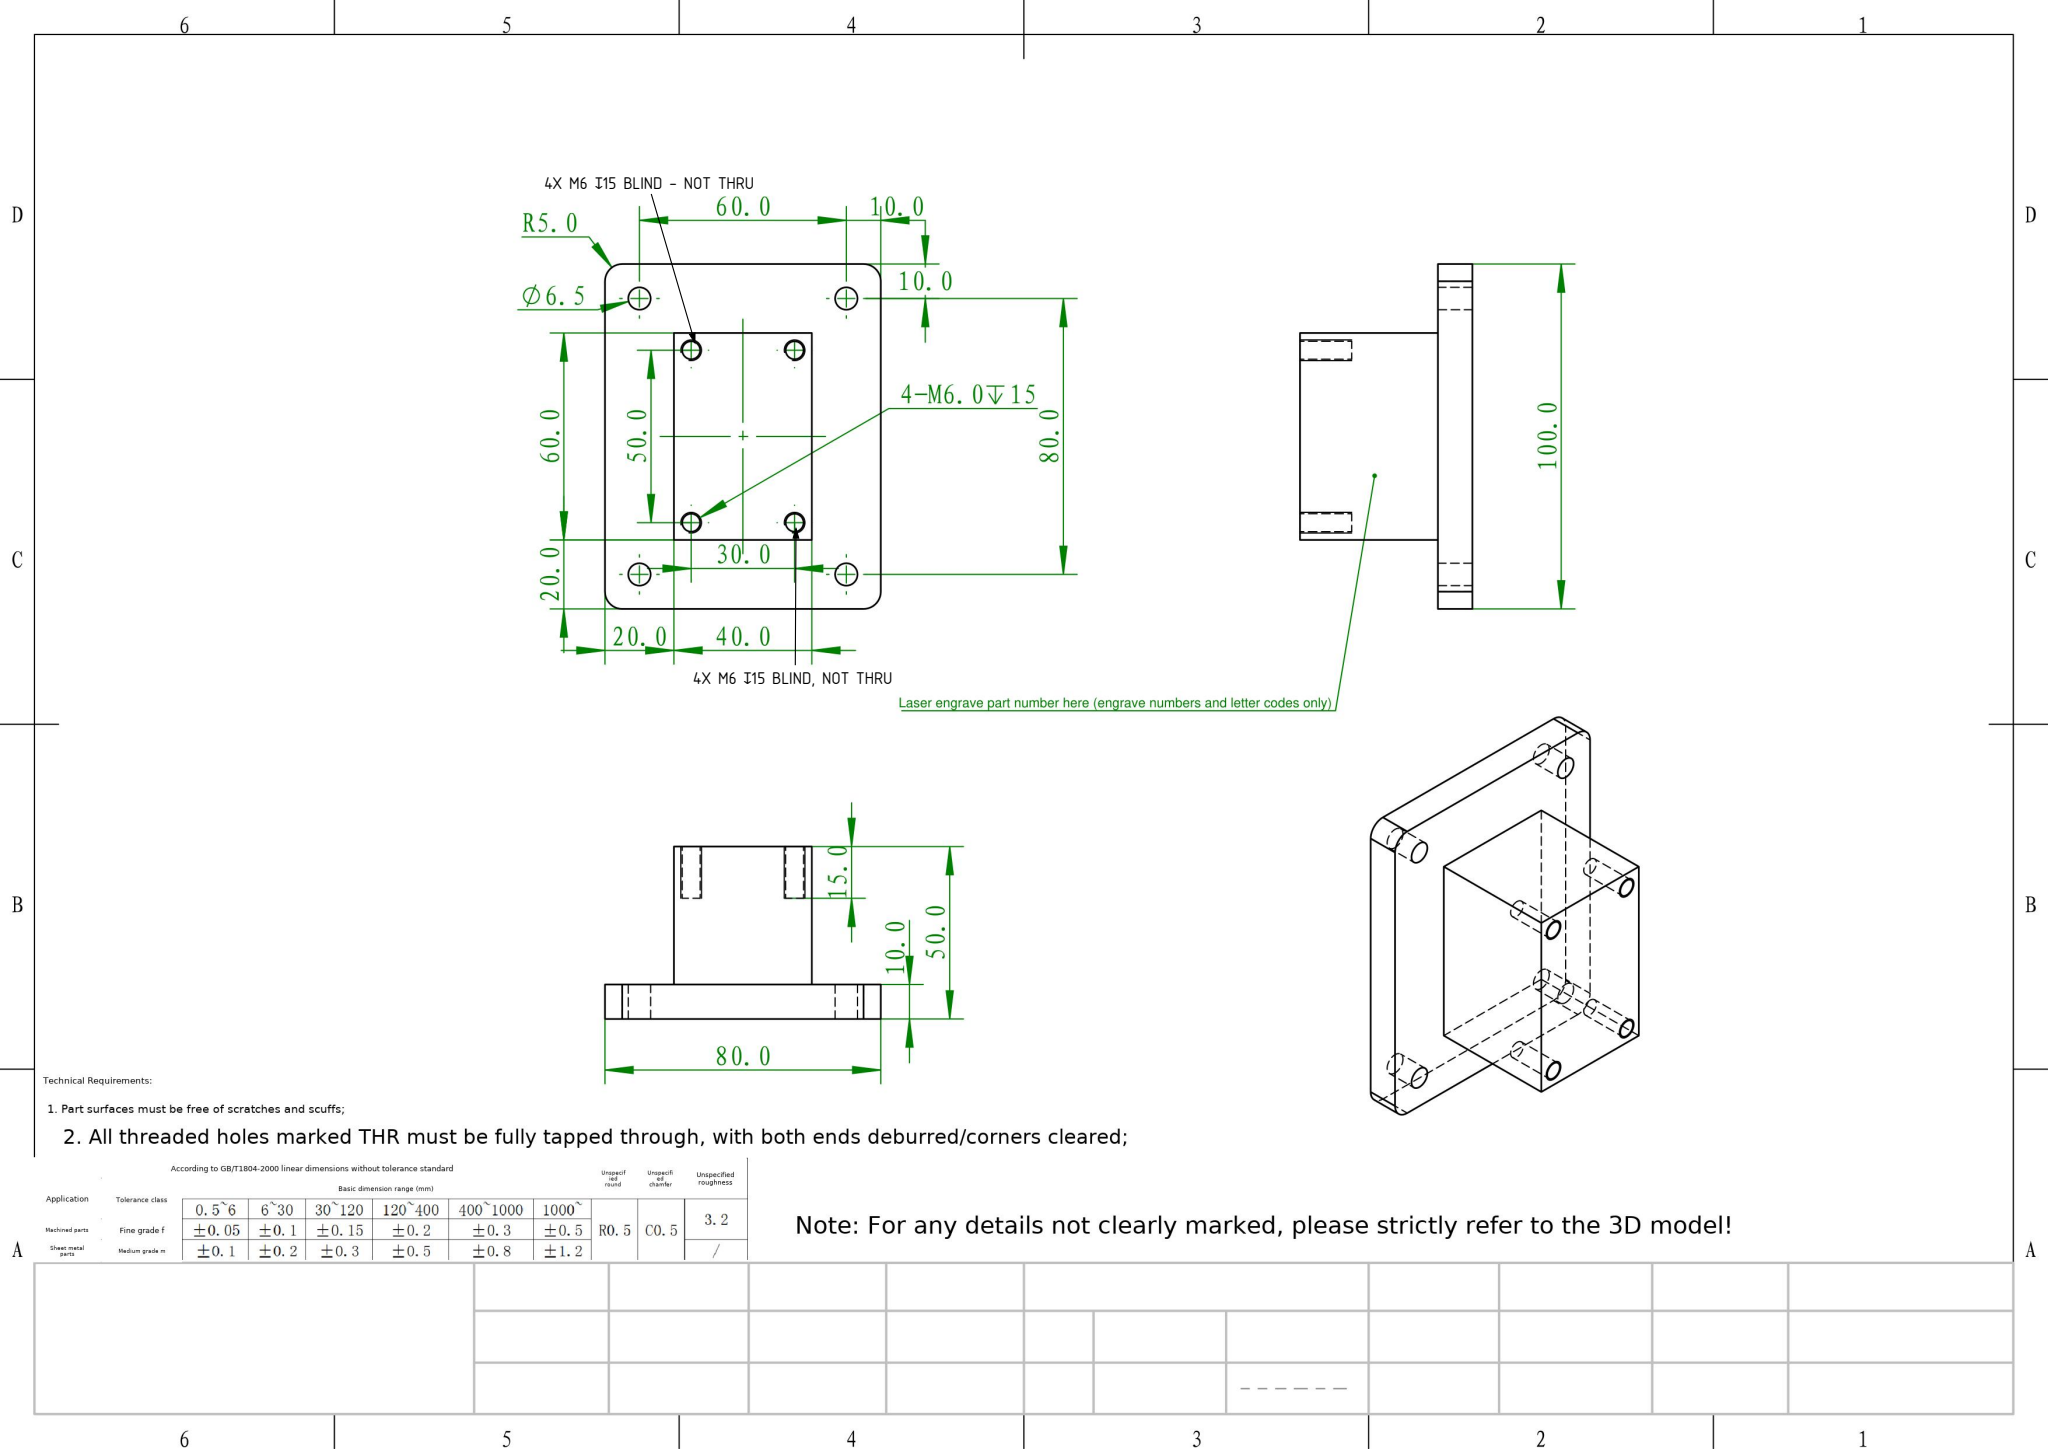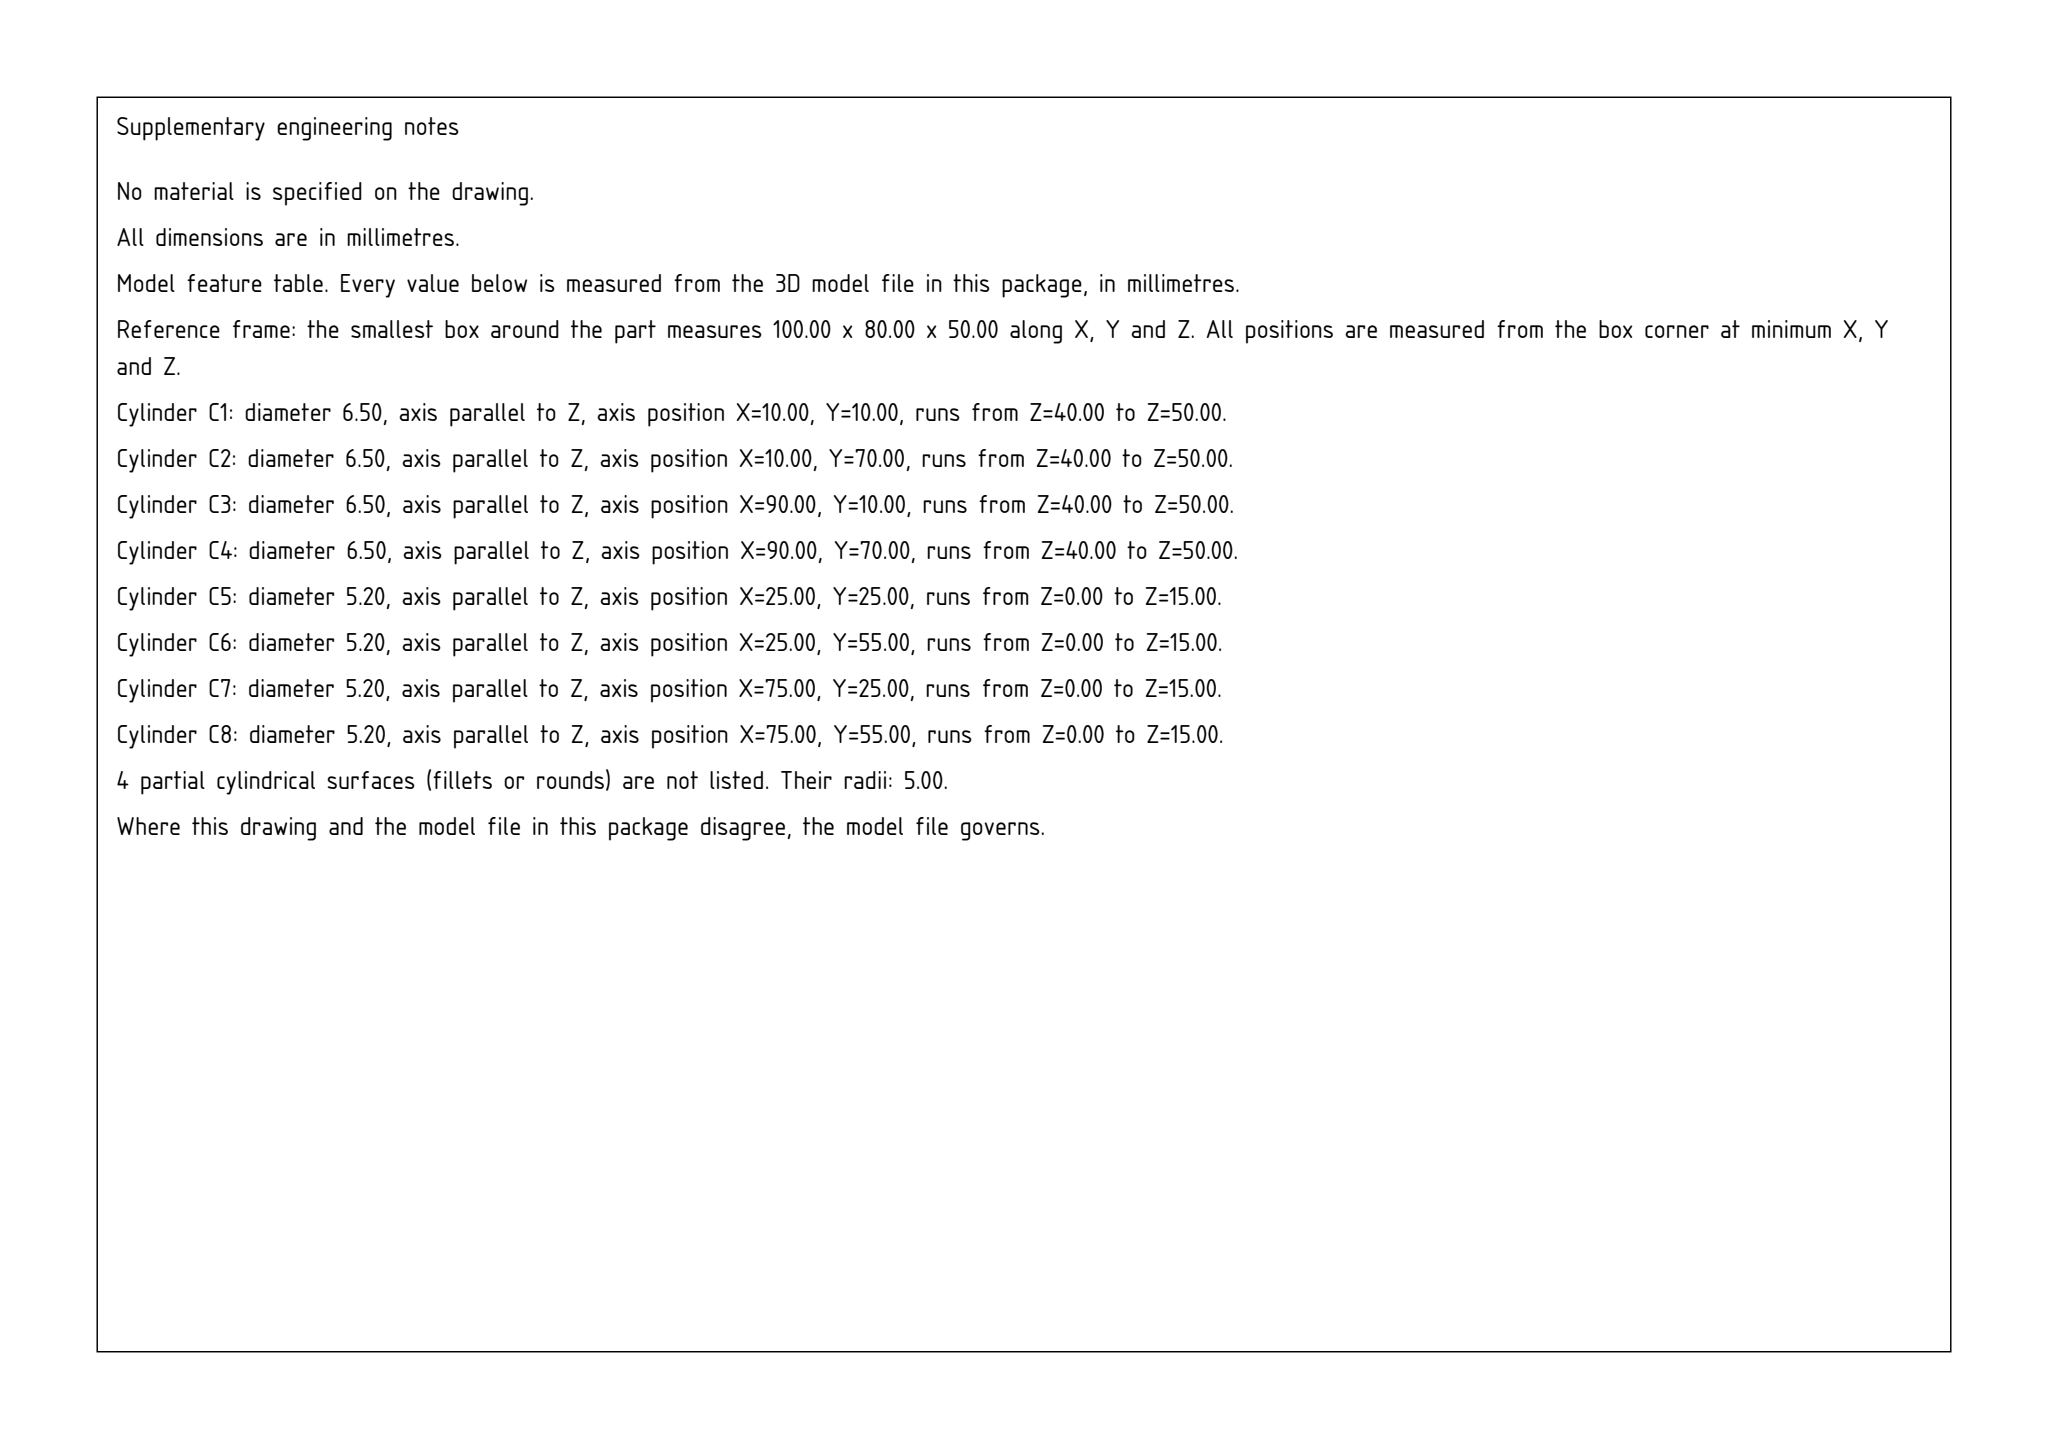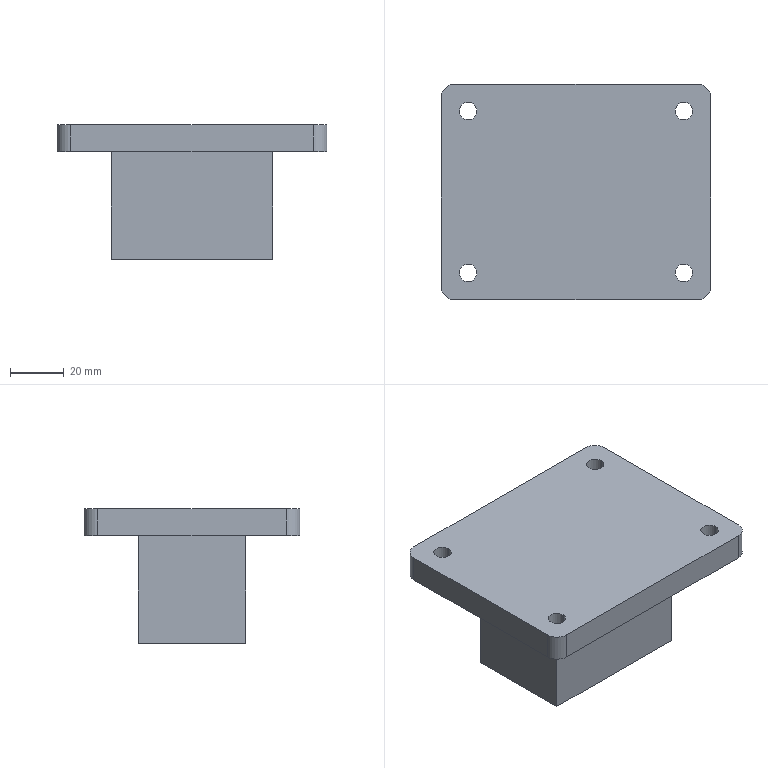Part | SolidWorks | mm | 1 solid | 35 faces | box 100 x 80 x 50 mm | volume 173184 mm3 | cylinder 20 | plane 15 | commonest cylinder face diameters 6.5 x8 5.2 x8 10 x4
Drawing notes:
4X M6 DP 15 BLIND IN BOSS END FACE - NOT THRU; DEBURR HOLE ENDS | from the solid: 4 holes dia 5.2 (M6 tap drill), axis z, at (25,25),(25,55),(75,25),(75,55), from z=0 to z=15 in boss spanning z=0..40; blind, flat bottom at z=15
4X M6 DP 15 BLIND FROM BOSS END FACE - NOT THRU; NO THR HOLES | from the solid: 4X holes ø5.2 axis z at (25,25),(25,55),(75,25),(75,55), from z=0 to z=15 with flat bottoms (z=15 faces, 21 mm² ea); boss spans z=0-40, so taps are blind, not through
build123d program:
from build123d import *

# Parameters (mm, degrees)
SKETCH1_W           = 60
SKETCH1_H           = 40
BOSS_EXTRUDE1_DEPTH = 40
SKETCH3_R           = 2.6
CUT_EXTRUDE2_DEPTH  = 15
SKETCH4_W           = 100
SKETCH4_H           = 80
BOSS_EXTRUDE2_DEPTH = 10
SKETCH5_R           = 3.25
CUT_EXTRUDE3_DEPTH  = 10
FILLET1_R           = 5


with BuildPart() as part:
    # Sketch1 → Boss-Extrude1 (new body)
    with BuildSketch(Plane.XY):
        Rectangle(SKETCH1_W, SKETCH1_H)
    extrude(amount=BOSS_EXTRUDE1_DEPTH)

    # Sketch3 → Cut-Extrude2 (cut)
    with BuildSketch(Plane(origin=(0, 0, 0), x_dir=(-1, 0, 0), z_dir=(0, 0, -1))):
        with Locations((-25, 15)):
            Circle(SKETCH3_R)
        with Locations((25, 15)):
            Circle(SKETCH3_R)
        with Locations((-25, -15)):
            Circle(SKETCH3_R)
        with Locations((25, -15)):
            Circle(SKETCH3_R)
    extrude(amount=-CUT_EXTRUDE2_DEPTH, mode=Mode.SUBTRACT)

    # Sketch4 → Boss-Extrude2 (add)
    with BuildSketch(Plane.XY.offset(40)):
        Rectangle(SKETCH4_W, SKETCH4_H)
    extrude(amount=BOSS_EXTRUDE2_DEPTH)

    # Sketch5 → Cut-Extrude3 (cut)
    with BuildSketch(Plane.XY.offset(50)):
        with Locations((-40, 30)):
            Circle(SKETCH5_R)
        with Locations((40, 30)):
            Circle(SKETCH5_R)
        with Locations((-40, -30)):
            Circle(SKETCH5_R)
        with Locations((40, -30)):
            Circle(SKETCH5_R)
    extrude(amount=-CUT_EXTRUDE3_DEPTH, mode=Mode.SUBTRACT)

    # Fillet1
    fillet1_edges = [part.edges().sort_by_distance(p)[0] for p in [
        (50, -40, 45),
        (50, 40, 45),
        (-50, 40, 45),
        (-50, -40, 45),
    ]]
    fillet(fillet1_edges, radius=FILLET1_R)


solid = part.part